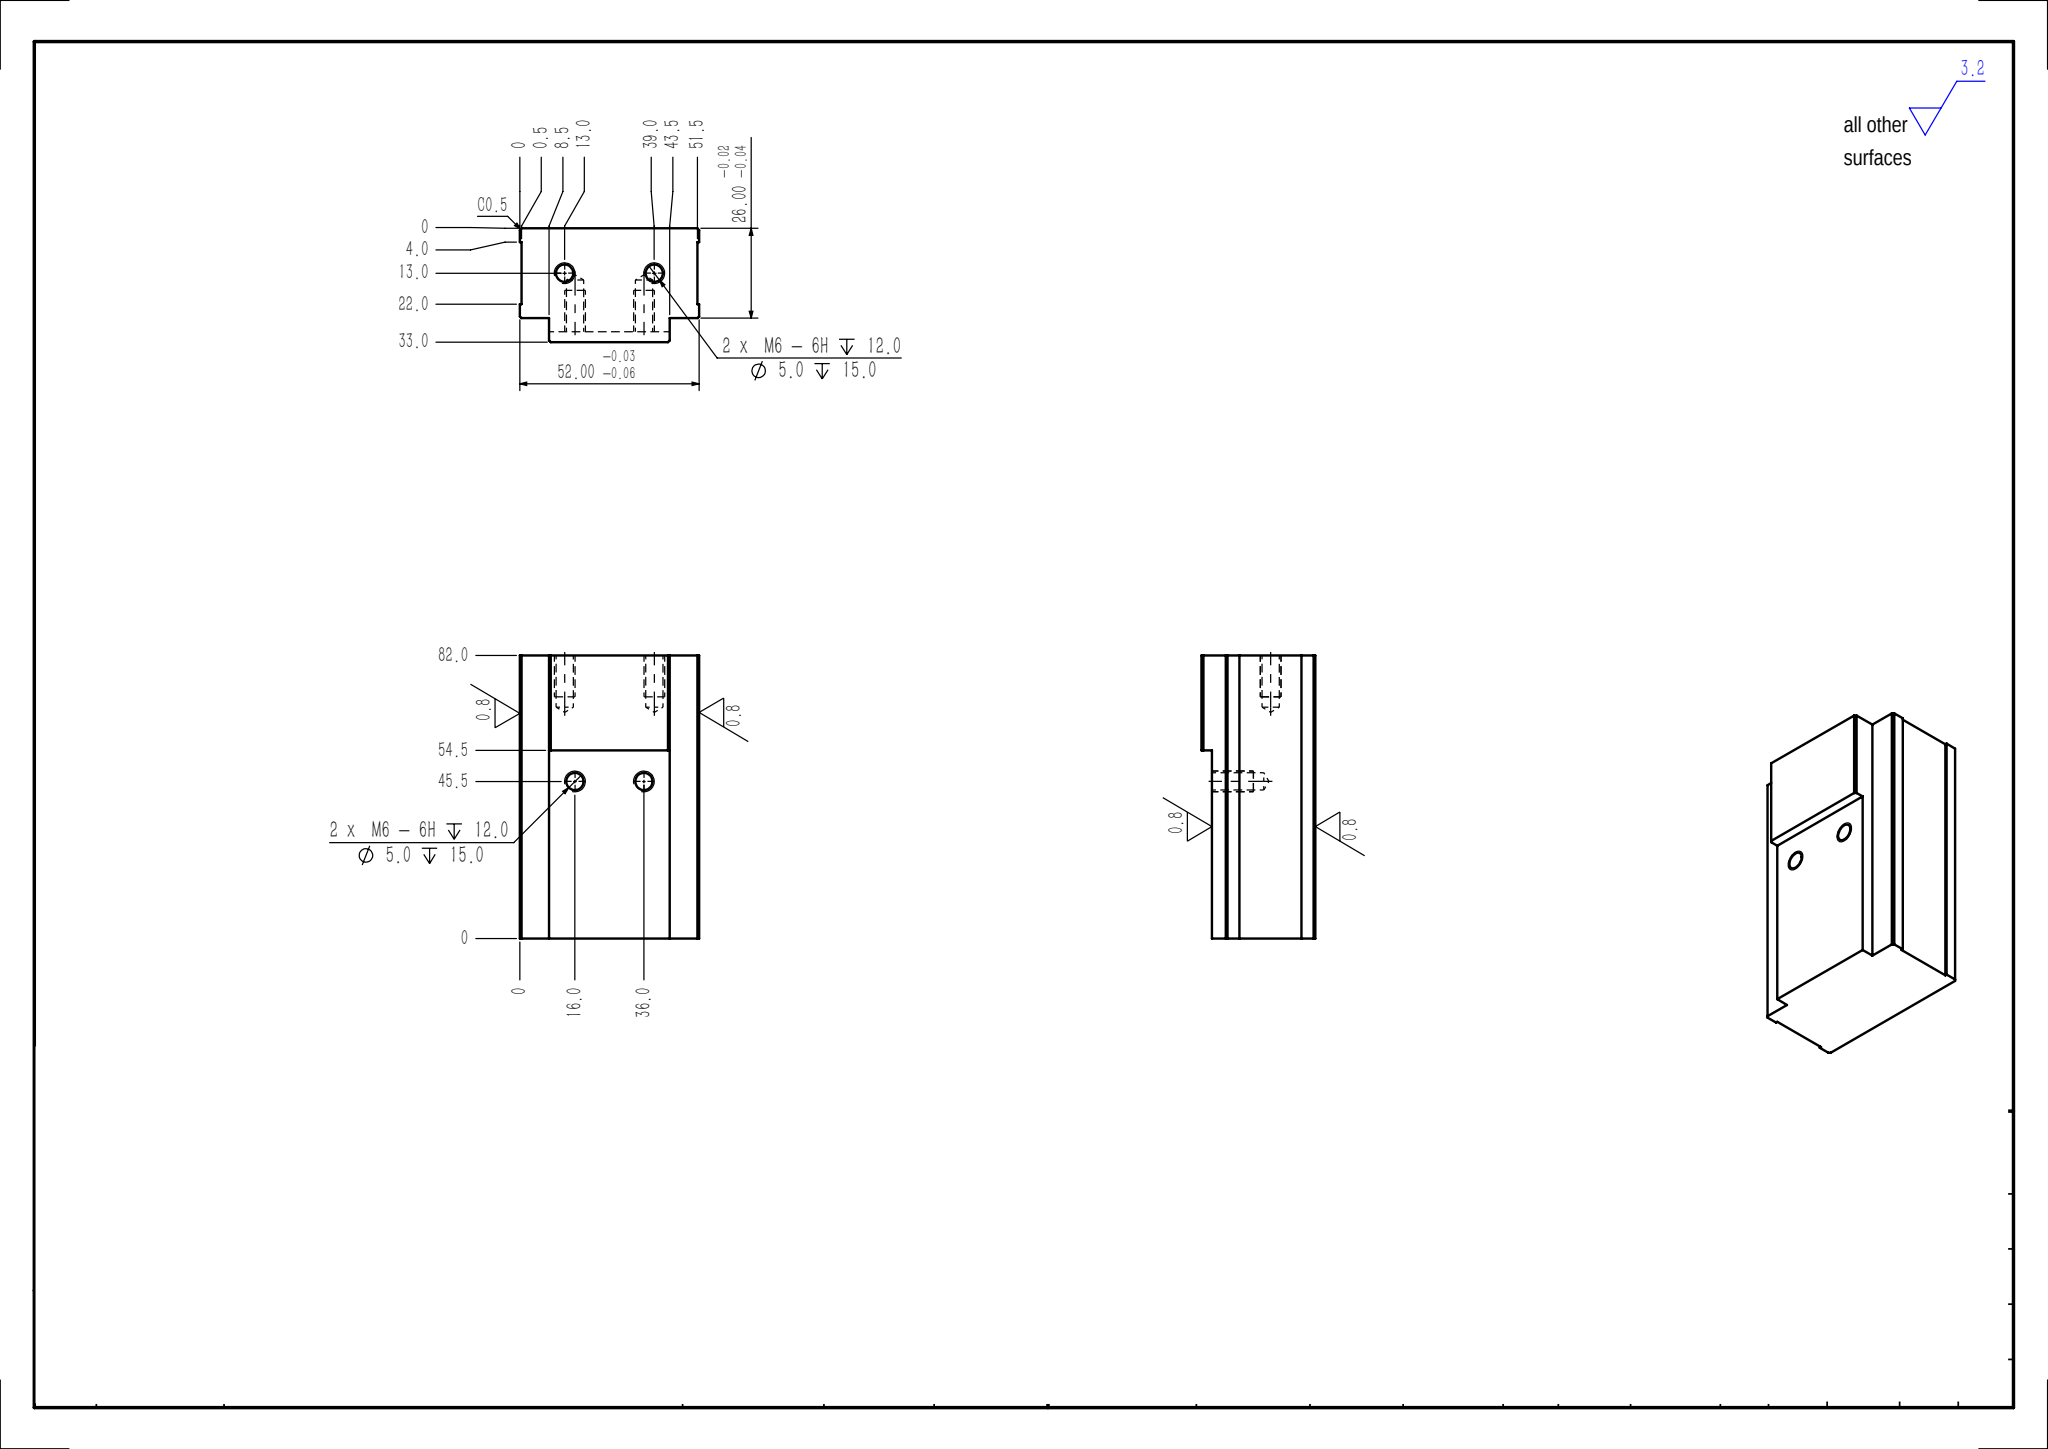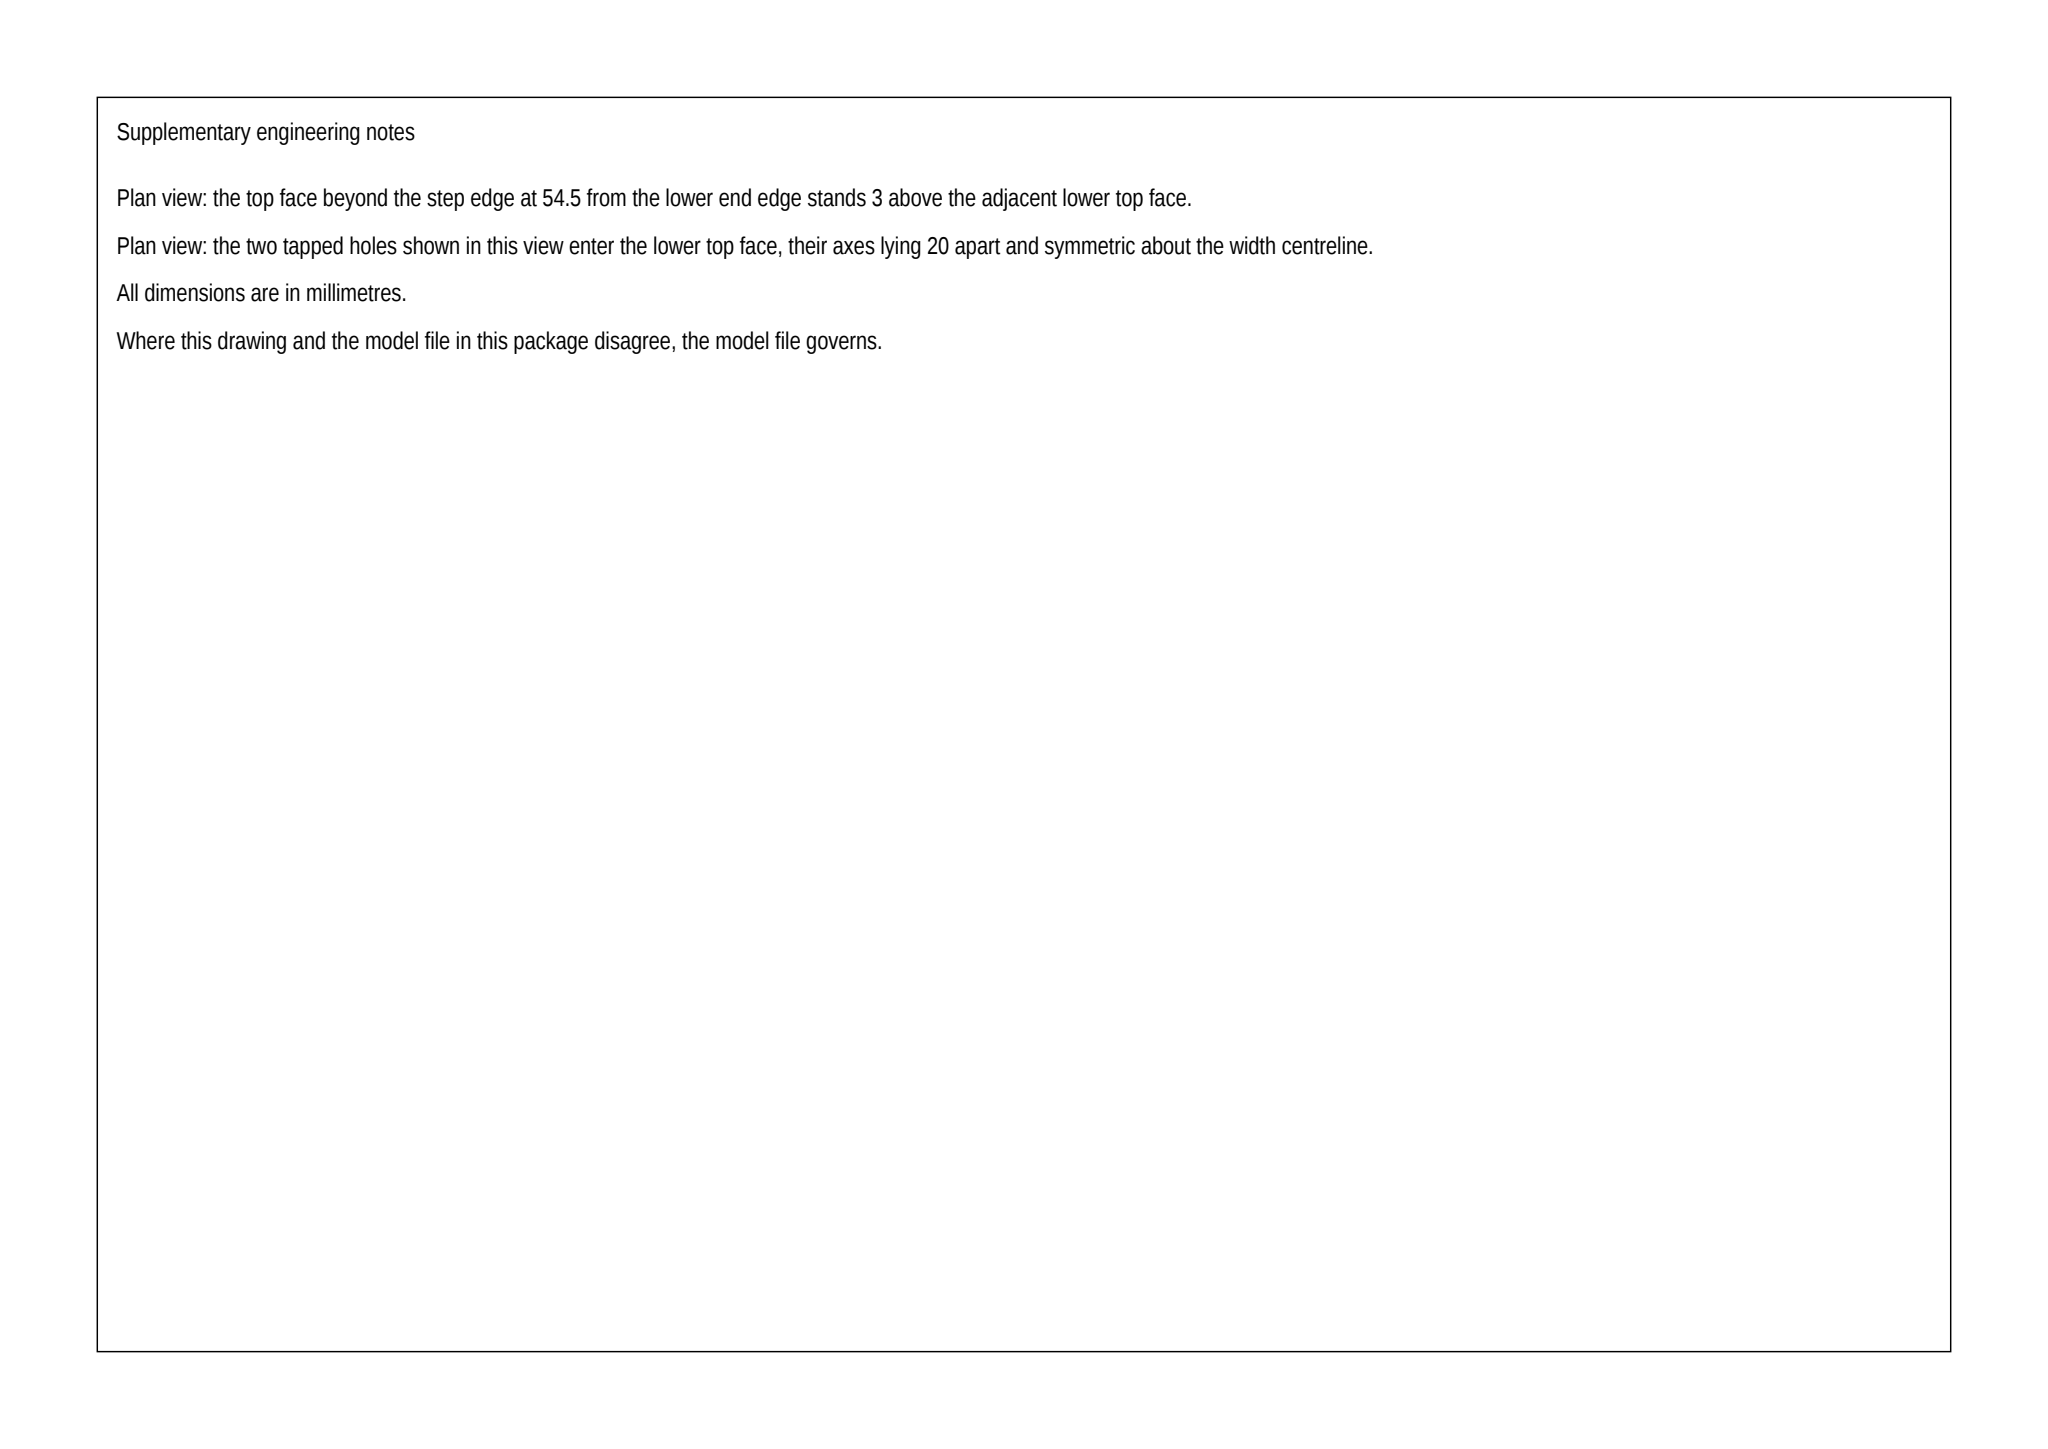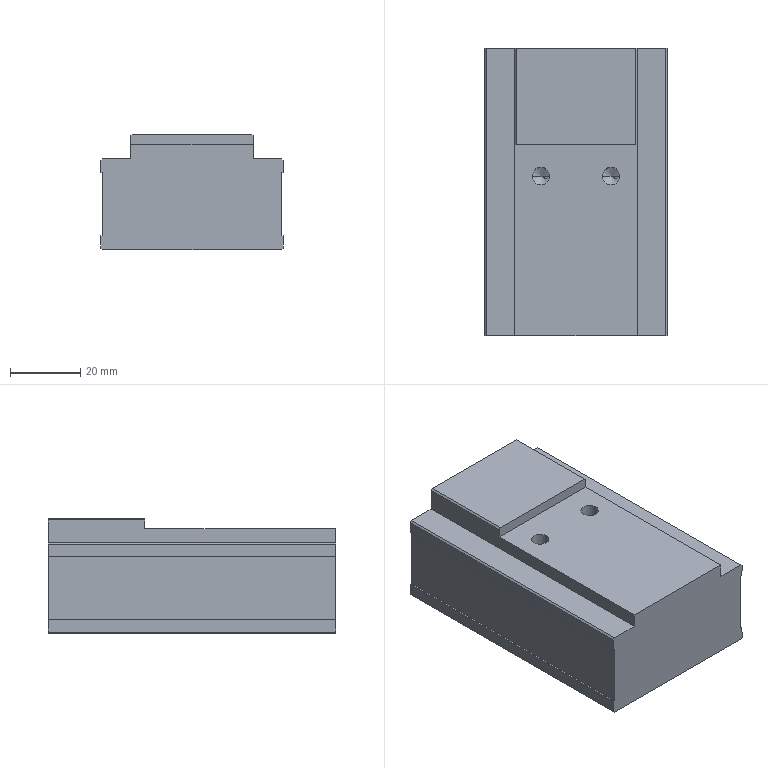Part | SolidWorks | mm | 1 solid | 42 faces | box 52 x 82 x 33 mm | volume 122490 mm3 | plane 26 | cylinder 8 | cone 8 | commonest cylinder face diameters 5 x8
build123d program:
from build123d import *

# Parameters (mm, degrees)
SKETCH1_W             = 52
SKETCH1_H             = 82
BOSS_EXTRUDE1_DEPTH   = 13
SKETCH2_W             = 35
SKETCH2_H             = 82
BOSS_EXTRUDE2_DEPTH   = 7
SKETCH3_W             = 35
SKETCH3_H             = 54.5
CUT_EXTRUDE1_DEPTH    = 3
M6_TAPPED_HOLE1_D     = 5
M6_TAPPED_HOLE1_DEPTH = 15
M6_TAPPED_HOLE1_TIP   = 1.502
CHAMFER1_SIZE         = 0.5
M6_TAPPED_HOLE2_D     = 5
M6_TAPPED_HOLE2_DEPTH = 15
M6_TAPPED_HOLE2_TIP   = 1.502
SKETCH9_W             = 18
SKETCH9_H             = 82
CUT_EXTRUDE3_DEPTH    = 0.5
SKETCH10_W            = 18
SKETCH10_H            = 82
CUT_EXTRUDE4_DEPTH    = 0.5


with BuildPart() as part:
    # Sketch1 → Boss-Extrude1 (new, symmetric)
    with BuildSketch(Plane.XY):
        Rectangle(SKETCH1_W, SKETCH1_H)
    extrude(amount=BOSS_EXTRUDE1_DEPTH, both=True)

    # Sketch2 → Boss-Extrude2 (add)
    with BuildSketch(Plane.XY.offset(13)):
        Rectangle(SKETCH2_W, SKETCH2_H)
    extrude(amount=BOSS_EXTRUDE2_DEPTH)

    # Sketch3 → Cut-Extrude1 (cut)
    with BuildSketch(Plane.XY.offset(20)):
        with Locations((0, -13.75)):
            Rectangle(SKETCH3_W, SKETCH3_H)
    extrude(amount=-CUT_EXTRUDE1_DEPTH, mode=Mode.SUBTRACT)

    # M6 Tapped Hole1
    with Locations(Plane.XY.offset(17)):
        with Locations((-10, 4.5), (10, 4.5)):
            Hole(M6_TAPPED_HOLE1_D / 2, depth=M6_TAPPED_HOLE1_DEPTH)
            with Locations((0, 0, -(M6_TAPPED_HOLE1_DEPTH + M6_TAPPED_HOLE1_TIP / 2))):  # 118° drill point
                Cone(0, M6_TAPPED_HOLE1_D / 2, M6_TAPPED_HOLE1_TIP, mode=Mode.SUBTRACT)

    # Chamfer1
    chamfer1_edges = [part.edges().sort_by_distance(p)[0] for p in [
        (-26, 0, 13),
        (-17.5, 27.25, 20),
        (17.5, 27.25, 20),
        (26, 0, 13),
        (-26, 0, -13),
        (26, 0, -13),
    ]]
    chamfer(chamfer1_edges, length=CHAMFER1_SIZE)

    # M6 Tapped Hole2
    with Locations(Plane(origin=(0, 41, 0), x_dir=(1, 0, 0), z_dir=(0, 1, 0))):
        with Locations((-13, 0), (13, 0)):
            Hole(M6_TAPPED_HOLE2_D / 2, depth=M6_TAPPED_HOLE2_DEPTH)
            with Locations((0, 0, -(M6_TAPPED_HOLE2_DEPTH + M6_TAPPED_HOLE2_TIP / 2))):  # 118° drill point
                Cone(0, M6_TAPPED_HOLE2_D / 2, M6_TAPPED_HOLE2_TIP, mode=Mode.SUBTRACT)

    # Sketch9 → Cut-Extrude3 (cut)
    with BuildSketch(Plane(origin=(26, 0, 0), x_dir=(0, 0, -1), z_dir=(1, 0, 0))):
        Rectangle(SKETCH9_W, SKETCH9_H)
    extrude(amount=-CUT_EXTRUDE3_DEPTH, mode=Mode.SUBTRACT)

    # Sketch10 → Cut-Extrude4 (cut)
    with BuildSketch(Plane.ZY.offset(26)):
        Rectangle(SKETCH10_W, SKETCH10_H)
    extrude(amount=-CUT_EXTRUDE4_DEPTH, mode=Mode.SUBTRACT)


solid = part.part